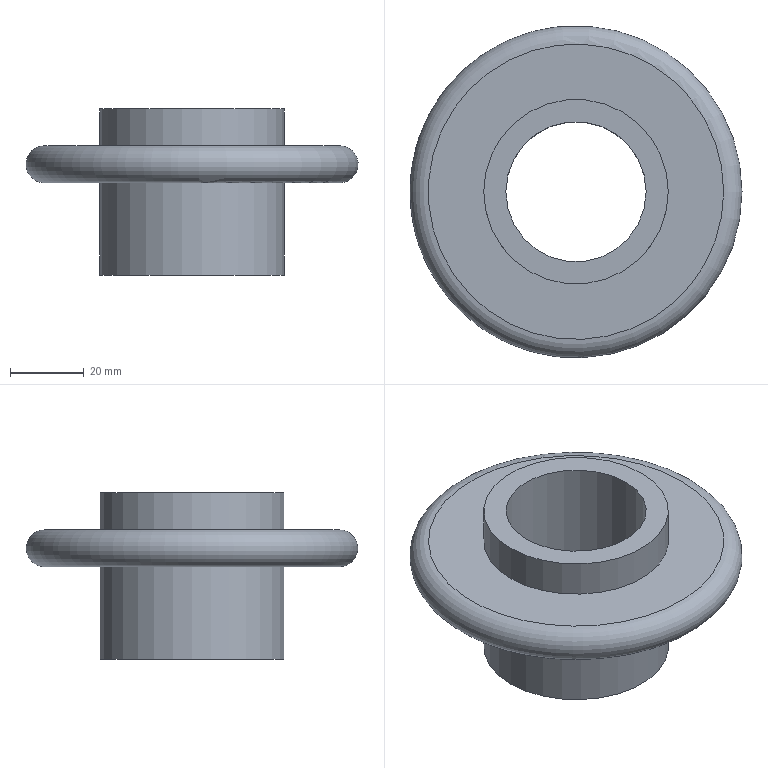Component | NX | NUT | 1 solid | 8 faces | box 90 x 90 x 45 mm | volume 78346 mm3 | plane 4 | cylinder 3 | torus 1 | commonest cylinder face diameters 50 x2 38 x1
STEP:
#1=CARTESIAN_POINT('',(0.,0.,0.));
#2=DIRECTION('',(0.,0.,1.));
#3=DIRECTION('',(1.,0.,0.));
#4=AXIS2_PLACEMENT_3D('',#1,#2,#3);
#5=CARTESIAN_POINT('',(-19.,240.,160.));
#6=VERTEX_POINT('',#5);
#7=CARTESIAN_POINT('',(0.,240.,160.));
#8=DIRECTION('',(0.,0.,-1.));
#9=DIRECTION('',(-1.,0.,0.));
#10=AXIS2_PLACEMENT_3D('',#7,#8,#9);
#11=CIRCLE('',#10,19.);
#12=CARTESIAN_POINT('',(0.,240.,160.));
#13=DIRECTION('',(0.,0.,-1.));
#14=DIRECTION('',(-1.,0.,0.));
#15=AXIS2_PLACEMENT_3D('',#12,#13,#14);
#16=CYLINDRICAL_SURFACE('',#15,19.);
#17=CARTESIAN_POINT('',(0.,0.));
#18=DIRECTION('',(1.,0.));
#19=VECTOR('',#18,1.);
#20=LINE('',#17,#19);
#21=(GEOMETRIC_REPRESENTATION_CONTEXT(2)PARAMETRIC_REPRESENTATION_CONTEXT()REPRESENTATION_CONTEXT('',''));
#22=DEFINITIONAL_REPRESENTATION('',(#20),#21);
#23=PCURVE('',#16,#22);
#24=CARTESIAN_POINT('',(0.,259.,160.));
#25=DIRECTION('',(0.,0.,-1.));
#26=DIRECTION('',(-1.,0.,0.));
#27=AXIS2_PLACEMENT_3D('',#24,#25,#26);
#28=PLANE('',#27);
#29=CARTESIAN_POINT('',(0.,-19.));
#30=DIRECTION('',(1.,0.));
#31=AXIS2_PLACEMENT_2D('',#29,#30);
#32=CIRCLE('',#31,19.);
#33=(GEOMETRIC_REPRESENTATION_CONTEXT(2)PARAMETRIC_REPRESENTATION_CONTEXT()REPRESENTATION_CONTEXT('',''));
#34=DEFINITIONAL_REPRESENTATION('',(#32),#33);
#35=PCURVE('',#28,#34);
#36=SURFACE_CURVE('',#11,(#23,#35),.PCURVE_S1.);
#37=EDGE_CURVE('',#6,#6,#36,.T.);
#38=ORIENTED_EDGE('',*,*,#37,.F.);
#39=CARTESIAN_POINT('',(-19.,240.,205.));
#40=VERTEX_POINT('',#39);
#41=CARTESIAN_POINT('',(-19.,240.,205.));
#42=CARTESIAN_POINT('',(-19.,240.,160.));
#43=B_SPLINE_CURVE_WITH_KNOTS('',1,(#41,#42),.UNSPECIFIED.,.F.,.F.,(2,2),(-45.,0.),.PIECEWISE_BEZIER_KNOTS.);
#44=CARTESIAN_POINT('',(0.,0.));
#45=DIRECTION('',(0.,1.));
#46=VECTOR('',#45,1.);
#47=LINE('',#44,#46);
#48=(GEOMETRIC_REPRESENTATION_CONTEXT(2)PARAMETRIC_REPRESENTATION_CONTEXT()REPRESENTATION_CONTEXT('',''));
#49=DEFINITIONAL_REPRESENTATION('',(#47),#48);
#50=PCURVE('',#16,#49);
#51=CARTESIAN_POINT('',(6.283,0.));
#52=DIRECTION('',(0.,1.));
#53=VECTOR('',#52,1.);
#54=LINE('',#51,#53);
#55=(GEOMETRIC_REPRESENTATION_CONTEXT(2)PARAMETRIC_REPRESENTATION_CONTEXT()REPRESENTATION_CONTEXT('',''));
#56=DEFINITIONAL_REPRESENTATION('',(#54),#55);
#57=PCURVE('',#16,#56);
#58=SEAM_CURVE('',#43,(#50,#57),.PCURVE_S1.);
#59=EDGE_CURVE('',#40,#6,#58,.T.);
#60=ORIENTED_EDGE('',*,*,#59,.F.);
#61=CARTESIAN_POINT('',(0.,240.,205.));
#62=DIRECTION('',(0.,0.,-1.));
#63=DIRECTION('',(-1.,0.,0.));
#64=AXIS2_PLACEMENT_3D('',#61,#62,#63);
#65=CIRCLE('',#64,19.);
#66=CARTESIAN_POINT('',(0.,-45.));
#67=DIRECTION('',(1.,0.));
#68=VECTOR('',#67,1.);
#69=LINE('',#66,#68);
#70=(GEOMETRIC_REPRESENTATION_CONTEXT(2)PARAMETRIC_REPRESENTATION_CONTEXT()REPRESENTATION_CONTEXT('',''));
#71=DEFINITIONAL_REPRESENTATION('',(#69),#70);
#72=PCURVE('',#16,#71);
#73=CARTESIAN_POINT('',(0.,265.,205.));
#74=DIRECTION('',(0.,0.,1.));
#75=DIRECTION('',(1.,0.,0.));
#76=AXIS2_PLACEMENT_3D('',#73,#74,#75);
#77=PLANE('',#76);
#78=CARTESIAN_POINT('',(-19.,-25.));
#79=CARTESIAN_POINT('',(-19.,7.909));
#80=CARTESIAN_POINT('',(9.5,-8.546));
#81=CARTESIAN_POINT('',(38.,-25.));
#82=CARTESIAN_POINT('',(9.5,-41.454));
#83=CARTESIAN_POINT('',(-19.,-57.909));
#84=CARTESIAN_POINT('',(-19.,-25.));
#85=(BOUNDED_CURVE()B_SPLINE_CURVE(2,(#78,#79,#80,#81,#82,#83,#84),.UNSPECIFIED.,.T.,.F.)B_SPLINE_CURVE_WITH_KNOTS((1,2,2,2,2,1),(-2.094,0.,2.094,4.189,6.283,8.378),.UNSPECIFIED.)CURVE()GEOMETRIC_REPRESENTATION_ITEM()RATIONAL_B_SPLINE_CURVE((1.,0.5,1.,0.5,1.,0.5,1.))REPRESENTATION_ITEM(''));
#86=(GEOMETRIC_REPRESENTATION_CONTEXT(2)PARAMETRIC_REPRESENTATION_CONTEXT()REPRESENTATION_CONTEXT('',''));
#87=DEFINITIONAL_REPRESENTATION('',(#85),#86);
#88=PCURVE('',#77,#87);
#89=SURFACE_CURVE('',#65,(#72,#88),.PCURVE_S1.);
#90=EDGE_CURVE('',#40,#40,#89,.T.);
#91=ORIENTED_EDGE('',*,*,#90,.T.);
#92=ORIENTED_EDGE('',*,*,#59,.T.);
#93=EDGE_LOOP('',(#38,#60,#91,#92));
#94=FACE_BOUND('',#93,.F.);
#95=ADVANCED_FACE('',(#94),#16,.F.);
#96=CARTESIAN_POINT('',(-25.,240.,160.));
#97=VERTEX_POINT('',#96);
#98=CARTESIAN_POINT('',(0.,240.,160.));
#99=DIRECTION('',(0.,0.,-1.));
#100=DIRECTION('',(-1.,0.,0.));
#101=AXIS2_PLACEMENT_3D('',#98,#99,#100);
#102=CIRCLE('',#101,25.);
#103=CARTESIAN_POINT('',(0.,-19.));
#104=DIRECTION('',(1.,0.));
#105=AXIS2_PLACEMENT_2D('',#103,#104);
#106=CIRCLE('',#105,25.);
#107=(GEOMETRIC_REPRESENTATION_CONTEXT(2)PARAMETRIC_REPRESENTATION_CONTEXT()REPRESENTATION_CONTEXT('',''));
#108=DEFINITIONAL_REPRESENTATION('',(#106),#107);
#109=PCURVE('',#28,#108);
#110=CARTESIAN_POINT('',(0.,240.,160.));
#111=DIRECTION('',(0.,0.,-1.));
#112=DIRECTION('',(-1.,0.,0.));
#113=AXIS2_PLACEMENT_3D('',#110,#111,#112);
#114=CYLINDRICAL_SURFACE('',#113,25.);
#115=CARTESIAN_POINT('',(0.,0.));
#116=DIRECTION('',(1.,0.));
#117=VECTOR('',#116,1.);
#118=LINE('',#115,#117);
#119=(GEOMETRIC_REPRESENTATION_CONTEXT(2)PARAMETRIC_REPRESENTATION_CONTEXT()REPRESENTATION_CONTEXT('',''));
#120=DEFINITIONAL_REPRESENTATION('',(#118),#119);
#121=PCURVE('',#114,#120);
#122=SURFACE_CURVE('',#102,(#109,#121),.PCURVE_S1.);
#123=EDGE_CURVE('',#97,#97,#122,.T.);
#124=ORIENTED_EDGE('',*,*,#123,.T.);
#125=EDGE_LOOP('',(#124));
#126=FACE_BOUND('',#125,.T.);
#127=ORIENTED_EDGE('',*,*,#37,.F.);
#128=EDGE_LOOP('',(#127));
#129=FACE_BOUND('',#128,.T.);
#130=ADVANCED_FACE('',(#126,#129),#28,.T.);
#131=CARTESIAN_POINT('',(-25.,240.,185.));
#132=VERTEX_POINT('',#131);
#133=CARTESIAN_POINT('',(0.,240.,185.));
#134=DIRECTION('',(0.,0.,-1.));
#135=DIRECTION('',(-1.,0.,0.));
#136=AXIS2_PLACEMENT_3D('',#133,#134,#135);
#137=CIRCLE('',#136,25.);
#138=CARTESIAN_POINT('',(0.,-25.));
#139=DIRECTION('',(1.,0.));
#140=VECTOR('',#139,1.);
#141=LINE('',#138,#140);
#142=(GEOMETRIC_REPRESENTATION_CONTEXT(2)PARAMETRIC_REPRESENTATION_CONTEXT()REPRESENTATION_CONTEXT('',''));
#143=DEFINITIONAL_REPRESENTATION('',(#141),#142);
#144=PCURVE('',#114,#143);
#145=CARTESIAN_POINT('',(0.,265.,185.));
#146=DIRECTION('',(0.,0.,-1.));
#147=DIRECTION('',(-1.,0.,0.));
#148=AXIS2_PLACEMENT_3D('',#145,#146,#147);
#149=PLANE('',#148);
#150=CARTESIAN_POINT('',(0.,-25.));
#151=DIRECTION('',(1.,0.));
#152=AXIS2_PLACEMENT_2D('',#150,#151);
#153=CIRCLE('',#152,25.);
#154=(GEOMETRIC_REPRESENTATION_CONTEXT(2)PARAMETRIC_REPRESENTATION_CONTEXT()REPRESENTATION_CONTEXT('',''));
#155=DEFINITIONAL_REPRESENTATION('',(#153),#154);
#156=PCURVE('',#149,#155);
#157=SURFACE_CURVE('',#137,(#144,#156),.PCURVE_S1.);
#158=EDGE_CURVE('',#132,#132,#157,.T.);
#159=ORIENTED_EDGE('',*,*,#158,.T.);
#160=CARTESIAN_POINT('',(-25.,240.,185.));
#161=CARTESIAN_POINT('',(-25.,240.,160.));
#162=B_SPLINE_CURVE_WITH_KNOTS('',1,(#160,#161),.UNSPECIFIED.,.F.,.F.,(2,2),(-25.,0.),.PIECEWISE_BEZIER_KNOTS.);
#163=CARTESIAN_POINT('',(6.283,0.));
#164=DIRECTION('',(0.,1.));
#165=VECTOR('',#164,1.);
#166=LINE('',#163,#165);
#167=(GEOMETRIC_REPRESENTATION_CONTEXT(2)PARAMETRIC_REPRESENTATION_CONTEXT()REPRESENTATION_CONTEXT('',''));
#168=DEFINITIONAL_REPRESENTATION('',(#166),#167);
#169=PCURVE('',#114,#168);
#170=CARTESIAN_POINT('',(0.,0.));
#171=DIRECTION('',(0.,1.));
#172=VECTOR('',#171,1.);
#173=LINE('',#170,#172);
#174=(GEOMETRIC_REPRESENTATION_CONTEXT(2)PARAMETRIC_REPRESENTATION_CONTEXT()REPRESENTATION_CONTEXT('',''));
#175=DEFINITIONAL_REPRESENTATION('',(#173),#174);
#176=PCURVE('',#114,#175);
#177=SEAM_CURVE('',#162,(#169,#176),.PCURVE_S1.);
#178=EDGE_CURVE('',#132,#97,#177,.T.);
#179=ORIENTED_EDGE('',*,*,#178,.T.);
#180=ORIENTED_EDGE('',*,*,#123,.F.);
#181=ORIENTED_EDGE('',*,*,#178,.F.);
#182=EDGE_LOOP('',(#159,#179,#180,#181));
#183=FACE_BOUND('',#182,.T.);
#184=ADVANCED_FACE('',(#183),#114,.T.);
#185=CARTESIAN_POINT('',(-40.,240.,185.));
#186=VERTEX_POINT('',#185);
#187=CARTESIAN_POINT('',(40.,240.,185.));
#188=VERTEX_POINT('',#187);
#189=CARTESIAN_POINT('',(0.,240.,185.));
#190=DIRECTION('',(0.,0.,-1.));
#191=DIRECTION('',(-1.,0.,0.));
#192=AXIS2_PLACEMENT_3D('',#189,#190,#191);
#193=CIRCLE('',#192,40.);
#194=CARTESIAN_POINT('',(0.,-25.));
#195=DIRECTION('',(1.,0.));
#196=AXIS2_PLACEMENT_2D('',#194,#195);
#197=CIRCLE('',#196,40.);
#198=(GEOMETRIC_REPRESENTATION_CONTEXT(2)PARAMETRIC_REPRESENTATION_CONTEXT()REPRESENTATION_CONTEXT('',''));
#199=DEFINITIONAL_REPRESENTATION('',(#197),#198);
#200=PCURVE('',#149,#199);
#201=CARTESIAN_POINT('',(0.,240.,190.));
#202=DIRECTION('',(0.,0.,1.));
#203=DIRECTION('',(1.,0.,0.));
#204=AXIS2_PLACEMENT_3D('',#201,#202,#203);
#205=TOROIDAL_SURFACE('',#204,40.,5.);
#206=CARTESIAN_POINT('',(3.142,4.712));
#207=DIRECTION('',(-1.,0.));
#208=VECTOR('',#207,1.);
#209=LINE('',#206,#208);
#210=(GEOMETRIC_REPRESENTATION_CONTEXT(2)PARAMETRIC_REPRESENTATION_CONTEXT()REPRESENTATION_CONTEXT('',''));
#211=DEFINITIONAL_REPRESENTATION('',(#209),#210);
#212=PCURVE('',#205,#211);
#213=SURFACE_CURVE('',#193,(#200,#212),.PCURVE_S1.);
#214=EDGE_CURVE('',#186,#188,#213,.T.);
#215=ORIENTED_EDGE('',*,*,#214,.T.);
#216=CARTESIAN_POINT('',(0.,240.,185.));
#217=DIRECTION('',(0.,0.,-1.));
#218=DIRECTION('',(-1.,0.,0.));
#219=AXIS2_PLACEMENT_3D('',#216,#217,#218);
#220=CIRCLE('',#219,40.);
#221=CARTESIAN_POINT('',(0.,-25.));
#222=DIRECTION('',(1.,0.));
#223=AXIS2_PLACEMENT_2D('',#221,#222);
#224=CIRCLE('',#223,40.);
#225=(GEOMETRIC_REPRESENTATION_CONTEXT(2)PARAMETRIC_REPRESENTATION_CONTEXT()REPRESENTATION_CONTEXT('',''));
#226=DEFINITIONAL_REPRESENTATION('',(#224),#225);
#227=PCURVE('',#149,#226);
#228=CARTESIAN_POINT('',(9.425,4.712));
#229=DIRECTION('',(-1.,0.));
#230=VECTOR('',#229,1.);
#231=LINE('',#228,#230);
#232=(GEOMETRIC_REPRESENTATION_CONTEXT(2)PARAMETRIC_REPRESENTATION_CONTEXT()REPRESENTATION_CONTEXT('',''));
#233=DEFINITIONAL_REPRESENTATION('',(#231),#232);
#234=PCURVE('',#205,#233);
#235=SURFACE_CURVE('',#220,(#227,#234),.PCURVE_S1.);
#236=EDGE_CURVE('',#188,#186,#235,.T.);
#237=ORIENTED_EDGE('',*,*,#236,.T.);
#238=EDGE_LOOP('',(#215,#237));
#239=FACE_BOUND('',#238,.T.);
#240=ORIENTED_EDGE('',*,*,#158,.F.);
#241=EDGE_LOOP('',(#240));
#242=FACE_BOUND('',#241,.T.);
#243=ADVANCED_FACE('',(#239,#242),#149,.T.);
#244=CARTESIAN_POINT('',(40.,240.,195.));
#245=VERTEX_POINT('',#244);
#246=CARTESIAN_POINT('',(0.,240.,195.));
#247=DIRECTION('',(0.,0.,1.));
#248=DIRECTION('',(1.,0.,0.));
#249=AXIS2_PLACEMENT_3D('',#246,#247,#248);
#250=CIRCLE('',#249,40.);
#251=CARTESIAN_POINT('',(0.,285.,195.));
#252=DIRECTION('',(0.,0.,1.));
#253=DIRECTION('',(1.,0.,0.));
#254=AXIS2_PLACEMENT_3D('',#251,#252,#253);
#255=PLANE('',#254);
#256=CARTESIAN_POINT('',(0.,-45.));
#257=DIRECTION('',(1.,0.));
#258=AXIS2_PLACEMENT_2D('',#256,#257);
#259=CIRCLE('',#258,40.);
#260=(GEOMETRIC_REPRESENTATION_CONTEXT(2)PARAMETRIC_REPRESENTATION_CONTEXT()REPRESENTATION_CONTEXT('',''));
#261=DEFINITIONAL_REPRESENTATION('',(#259),#260);
#262=PCURVE('',#255,#261);
#263=CARTESIAN_POINT('',(0.,7.854));
#264=DIRECTION('',(1.,0.));
#265=VECTOR('',#264,1.);
#266=LINE('',#263,#265);
#267=(GEOMETRIC_REPRESENTATION_CONTEXT(2)PARAMETRIC_REPRESENTATION_CONTEXT()REPRESENTATION_CONTEXT('',''));
#268=DEFINITIONAL_REPRESENTATION('',(#266),#267);
#269=PCURVE('',#205,#268);
#270=SURFACE_CURVE('',#250,(#262,#269),.PCURVE_S1.);
#271=EDGE_CURVE('',#245,#245,#270,.T.);
#272=ORIENTED_EDGE('',*,*,#271,.T.);
#273=EDGE_LOOP('',(#272));
#274=FACE_BOUND('',#273,.T.);
#275=CARTESIAN_POINT('',(-25.,240.,195.));
#276=VERTEX_POINT('',#275);
#277=CARTESIAN_POINT('',(0.,240.,195.));
#278=DIRECTION('',(0.,0.,-1.));
#279=DIRECTION('',(-1.,0.,0.));
#280=AXIS2_PLACEMENT_3D('',#277,#278,#279);
#281=CIRCLE('',#280,25.);
#282=CARTESIAN_POINT('',(-25.,-45.));
#283=CARTESIAN_POINT('',(-25.,-1.699));
#284=CARTESIAN_POINT('',(12.5,-23.349));
#285=CARTESIAN_POINT('',(50.,-45.));
#286=CARTESIAN_POINT('',(12.5,-66.651));
#287=CARTESIAN_POINT('',(-25.,-88.301));
#288=CARTESIAN_POINT('',(-25.,-45.));
#289=(BOUNDED_CURVE()B_SPLINE_CURVE(2,(#282,#283,#284,#285,#286,#287,#288),.UNSPECIFIED.,.T.,.F.)B_SPLINE_CURVE_WITH_KNOTS((1,2,2,2,2,1),(-2.094,0.,2.094,4.189,6.283,8.378),.UNSPECIFIED.)CURVE()GEOMETRIC_REPRESENTATION_ITEM()RATIONAL_B_SPLINE_CURVE((1.,0.5,1.,0.5,1.,0.5,1.))REPRESENTATION_ITEM(''));
#290=(GEOMETRIC_REPRESENTATION_CONTEXT(2)PARAMETRIC_REPRESENTATION_CONTEXT()REPRESENTATION_CONTEXT('',''));
#291=DEFINITIONAL_REPRESENTATION('',(#289),#290);
#292=PCURVE('',#255,#291);
#293=CARTESIAN_POINT('',(0.,240.,160.));
#294=DIRECTION('',(0.,0.,-1.));
#295=DIRECTION('',(-1.,0.,0.));
#296=AXIS2_PLACEMENT_3D('',#293,#294,#295);
#297=CYLINDRICAL_SURFACE('',#296,25.);
#298=CARTESIAN_POINT('',(0.,-35.));
#299=DIRECTION('',(1.,0.));
#300=VECTOR('',#299,1.);
#301=LINE('',#298,#300);
#302=(GEOMETRIC_REPRESENTATION_CONTEXT(2)PARAMETRIC_REPRESENTATION_CONTEXT()REPRESENTATION_CONTEXT('',''));
#303=DEFINITIONAL_REPRESENTATION('',(#301),#302);
#304=PCURVE('',#297,#303);
#305=SURFACE_CURVE('',#281,(#292,#304),.PCURVE_S1.);
#306=EDGE_CURVE('',#276,#276,#305,.T.);
#307=ORIENTED_EDGE('',*,*,#306,.T.);
#308=EDGE_LOOP('',(#307));
#309=FACE_BOUND('',#308,.T.);
#310=ADVANCED_FACE('',(#274,#309),#255,.T.);
#311=CARTESIAN_POINT('',(-25.,240.,205.));
#312=VERTEX_POINT('',#311);
#313=CARTESIAN_POINT('',(0.,240.,205.));
#314=DIRECTION('',(0.,0.,-1.));
#315=DIRECTION('',(-1.,0.,0.));
#316=AXIS2_PLACEMENT_3D('',#313,#314,#315);
#317=CIRCLE('',#316,25.);
#318=CARTESIAN_POINT('',(0.,-45.));
#319=DIRECTION('',(1.,0.));
#320=VECTOR('',#319,1.);
#321=LINE('',#318,#320);
#322=(GEOMETRIC_REPRESENTATION_CONTEXT(2)PARAMETRIC_REPRESENTATION_CONTEXT()REPRESENTATION_CONTEXT('',''));
#323=DEFINITIONAL_REPRESENTATION('',(#321),#322);
#324=PCURVE('',#297,#323);
#325=CARTESIAN_POINT('',(-25.,-25.));
#326=CARTESIAN_POINT('',(-25.,18.301));
#327=CARTESIAN_POINT('',(12.5,-3.349));
#328=CARTESIAN_POINT('',(50.,-25.));
#329=CARTESIAN_POINT('',(12.5,-46.651));
#330=CARTESIAN_POINT('',(-25.,-68.301));
#331=CARTESIAN_POINT('',(-25.,-25.));
#332=(BOUNDED_CURVE()B_SPLINE_CURVE(2,(#325,#326,#327,#328,#329,#330,#331),.UNSPECIFIED.,.T.,.F.)B_SPLINE_CURVE_WITH_KNOTS((1,2,2,2,2,1),(-2.094,0.,2.094,4.189,6.283,8.378),.UNSPECIFIED.)CURVE()GEOMETRIC_REPRESENTATION_ITEM()RATIONAL_B_SPLINE_CURVE((1.,0.5,1.,0.5,1.,0.5,1.))REPRESENTATION_ITEM(''));
#333=(GEOMETRIC_REPRESENTATION_CONTEXT(2)PARAMETRIC_REPRESENTATION_CONTEXT()REPRESENTATION_CONTEXT('',''));
#334=DEFINITIONAL_REPRESENTATION('',(#332),#333);
#335=PCURVE('',#77,#334);
#336=SURFACE_CURVE('',#317,(#324,#335),.PCURVE_S1.);
#337=EDGE_CURVE('',#312,#312,#336,.T.);
#338=ORIENTED_EDGE('',*,*,#337,.T.);
#339=CARTESIAN_POINT('',(-25.,240.,205.));
#340=CARTESIAN_POINT('',(-25.,240.,195.));
#341=B_SPLINE_CURVE_WITH_KNOTS('',1,(#339,#340),.UNSPECIFIED.,.F.,.F.,(2,2),(-45.,-35.),.PIECEWISE_BEZIER_KNOTS.);
#342=CARTESIAN_POINT('',(6.283,0.));
#343=DIRECTION('',(0.,1.));
#344=VECTOR('',#343,1.);
#345=LINE('',#342,#344);
#346=(GEOMETRIC_REPRESENTATION_CONTEXT(2)PARAMETRIC_REPRESENTATION_CONTEXT()REPRESENTATION_CONTEXT('',''));
#347=DEFINITIONAL_REPRESENTATION('',(#345),#346);
#348=PCURVE('',#297,#347);
#349=CARTESIAN_POINT('',(0.,0.));
#350=DIRECTION('',(0.,1.));
#351=VECTOR('',#350,1.);
#352=LINE('',#349,#351);
#353=(GEOMETRIC_REPRESENTATION_CONTEXT(2)PARAMETRIC_REPRESENTATION_CONTEXT()REPRESENTATION_CONTEXT('',''));
#354=DEFINITIONAL_REPRESENTATION('',(#352),#353);
#355=PCURVE('',#297,#354);
#356=SEAM_CURVE('',#341,(#348,#355),.PCURVE_S1.);
#357=EDGE_CURVE('',#312,#276,#356,.T.);
#358=ORIENTED_EDGE('',*,*,#357,.T.);
#359=ORIENTED_EDGE('',*,*,#306,.F.);
#360=ORIENTED_EDGE('',*,*,#357,.F.);
#361=EDGE_LOOP('',(#338,#358,#359,#360));
#362=FACE_BOUND('',#361,.T.);
#363=ADVANCED_FACE('',(#362),#297,.T.);
#364=ORIENTED_EDGE('',*,*,#90,.T.);
#365=EDGE_LOOP('',(#364));
#366=FACE_BOUND('',#365,.T.);
#367=ORIENTED_EDGE('',*,*,#337,.F.);
#368=EDGE_LOOP('',(#367));
#369=FACE_BOUND('',#368,.T.);
#370=ADVANCED_FACE('',(#366,#369),#77,.T.);
#371=ORIENTED_EDGE('',*,*,#271,.F.);
#372=CARTESIAN_POINT('',(40.,240.,185.));
#373=CARTESIAN_POINT('',(41.963,240.,185.));
#374=CARTESIAN_POINT('',(43.927,240.,185.881));
#375=CARTESIAN_POINT('',(45.429,240.,187.643));
#376=CARTESIAN_POINT('',(46.009,240.,190.));
#377=CARTESIAN_POINT('',(45.429,240.,192.357));
#378=CARTESIAN_POINT('',(43.927,240.,194.119));
#379=CARTESIAN_POINT('',(41.963,240.,195.));
#380=CARTESIAN_POINT('',(40.,240.,195.));
#381=B_SPLINE_CURVE_WITH_KNOTS('',8,(#372,#373,#374,#375,#376,#377,#378,#379,#380),.UNSPECIFIED.,.F.,.F.,(9,9),(-1.571,1.571),.PIECEWISE_BEZIER_KNOTS.);
#382=CARTESIAN_POINT('',(0.,6.283));
#383=DIRECTION('',(0.,1.));
#384=VECTOR('',#383,1.);
#385=LINE('',#382,#384);
#386=(GEOMETRIC_REPRESENTATION_CONTEXT(2)PARAMETRIC_REPRESENTATION_CONTEXT()REPRESENTATION_CONTEXT('',''));
#387=DEFINITIONAL_REPRESENTATION('',(#385),#386);
#388=PCURVE('',#205,#387);
#389=CARTESIAN_POINT('',(6.283,6.283));
#390=DIRECTION('',(0.,1.));
#391=VECTOR('',#390,1.);
#392=LINE('',#389,#391);
#393=(GEOMETRIC_REPRESENTATION_CONTEXT(2)PARAMETRIC_REPRESENTATION_CONTEXT()REPRESENTATION_CONTEXT('',''));
#394=DEFINITIONAL_REPRESENTATION('',(#392),#393);
#395=PCURVE('',#205,#394);
#396=SEAM_CURVE('',#381,(#388,#395),.PCURVE_S1.);
#397=EDGE_CURVE('',#188,#245,#396,.T.);
#398=ORIENTED_EDGE('',*,*,#397,.F.);
#399=ORIENTED_EDGE('',*,*,#214,.F.);
#400=ORIENTED_EDGE('',*,*,#236,.F.);
#401=ORIENTED_EDGE('',*,*,#397,.T.);
#402=EDGE_LOOP('',(#371,#398,#399,#400,#401));
#403=FACE_BOUND('',#402,.T.);
#404=ADVANCED_FACE('',(#403),#205,.T.);
#405=CLOSED_SHELL('',(#95,#130,#184,#243,#310,#363,#370,#404));
#406=MANIFOLD_SOLID_BREP('',#405);
#407=(LENGTH_UNIT()NAMED_UNIT(*)SI_UNIT(.MILLI.,.METRE.));
#408=UNCERTAINTY_MEASURE_WITH_UNIT(LENGTH_MEASURE(0.000005),#407,'','');
#409=(NAMED_UNIT(*)PLANE_ANGLE_UNIT()SI_UNIT($,.RADIAN.));
#410=(NAMED_UNIT(*)SI_UNIT($,.STERADIAN.)SOLID_ANGLE_UNIT());
#411=(GEOMETRIC_REPRESENTATION_CONTEXT(3)GLOBAL_UNCERTAINTY_ASSIGNED_CONTEXT((#408))GLOBAL_UNIT_ASSIGNED_CONTEXT((#407,#409,#410))REPRESENTATION_CONTEXT('',''));
#412=ADVANCED_BREP_SHAPE_REPRESENTATION('',(#4,#406),#411);